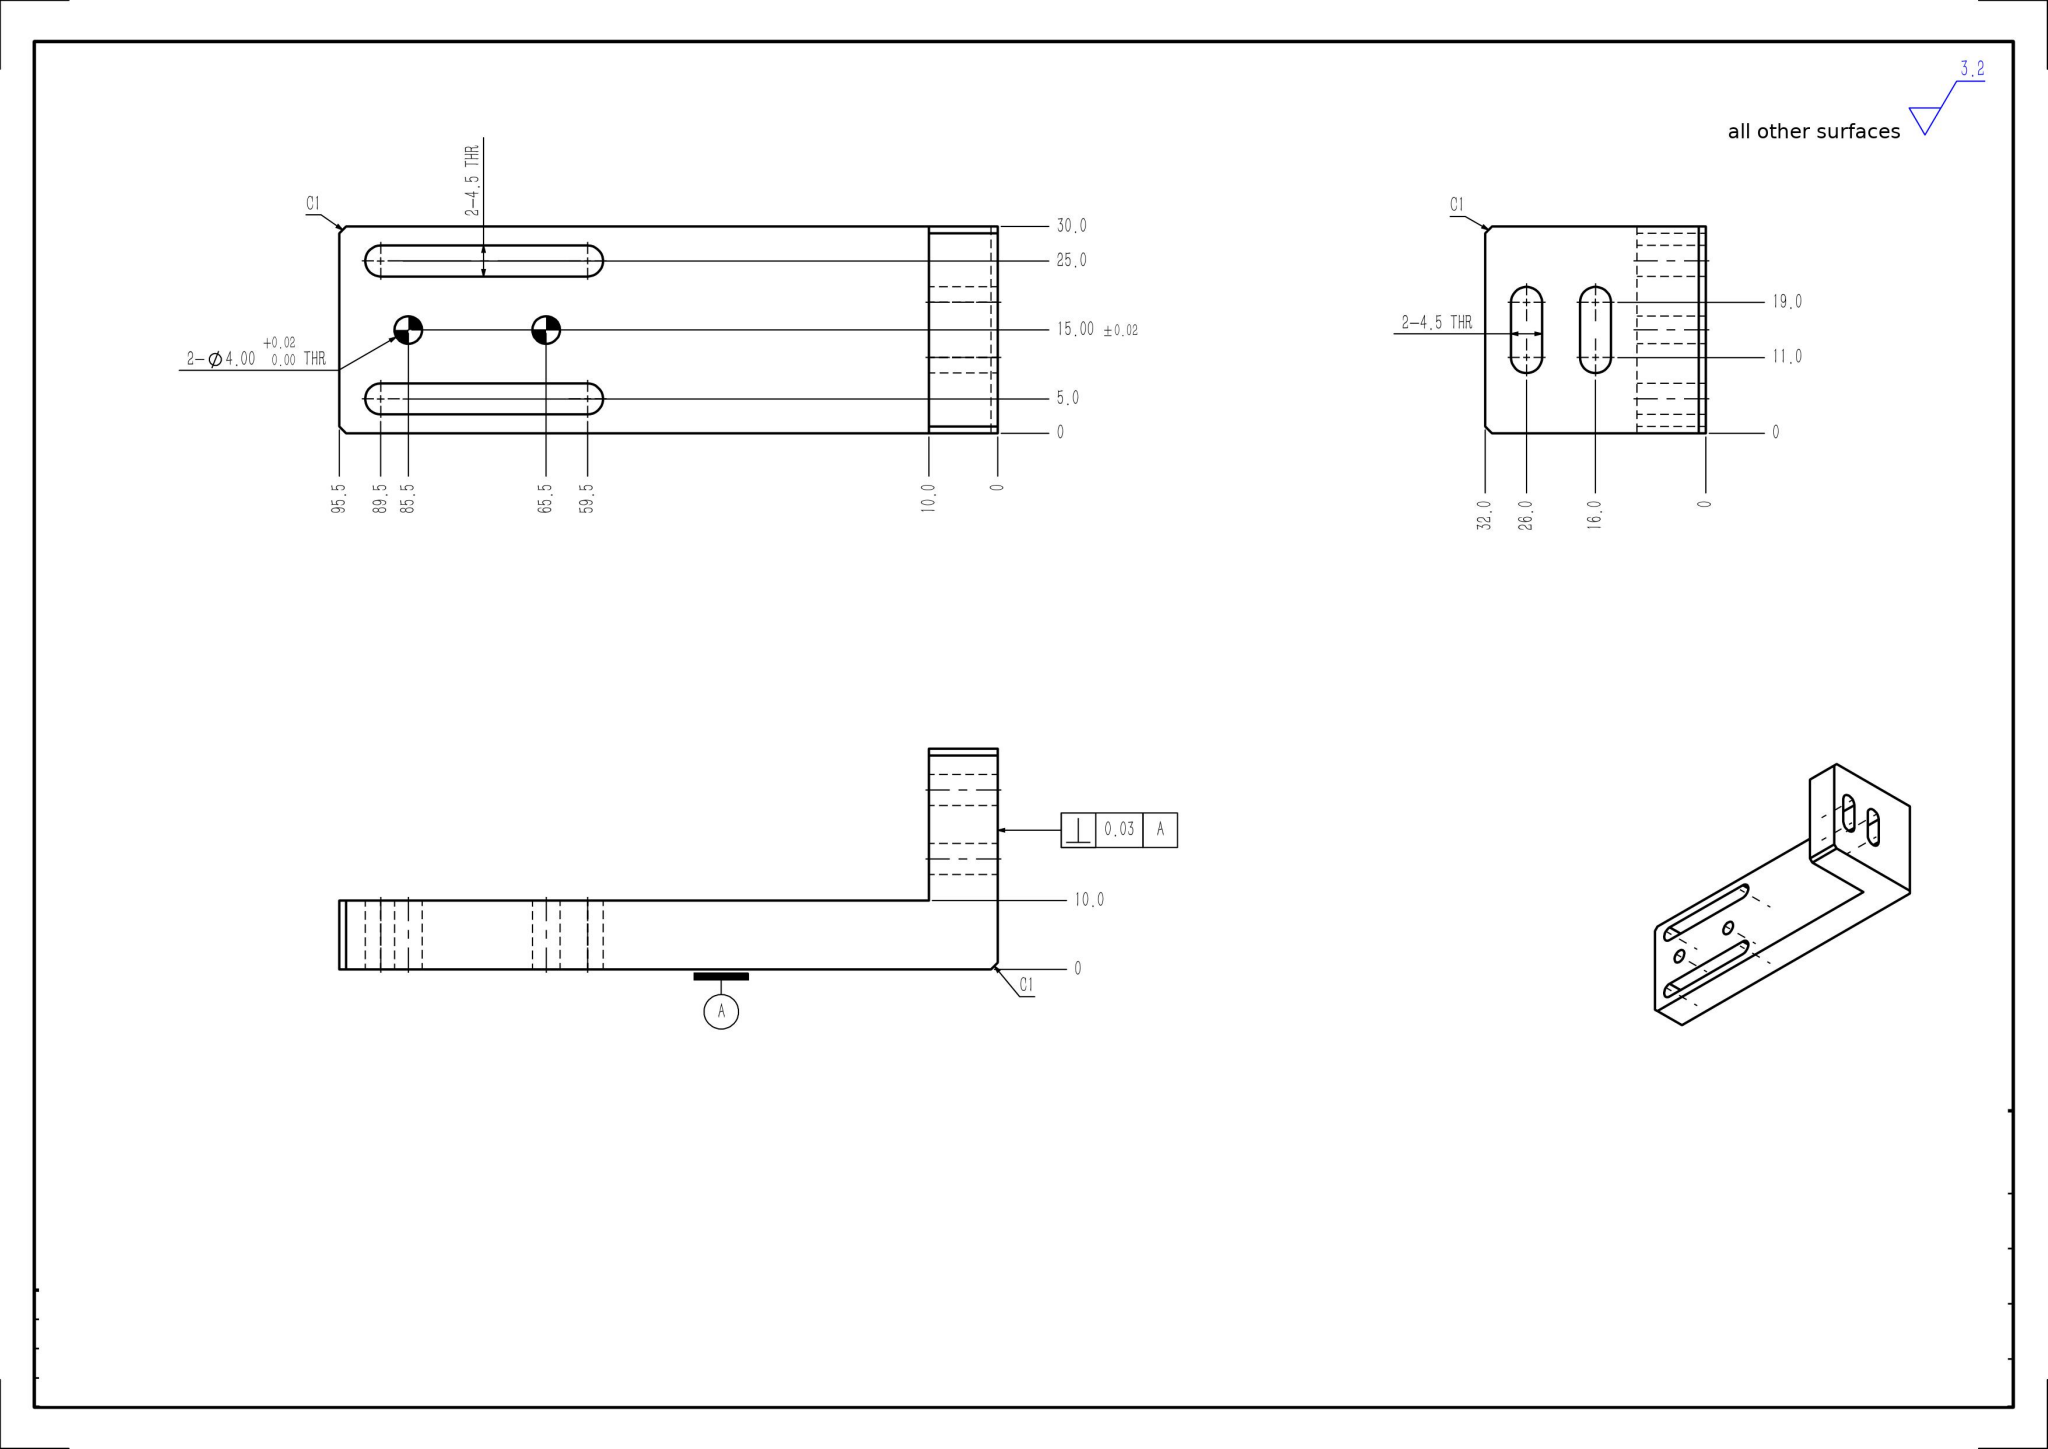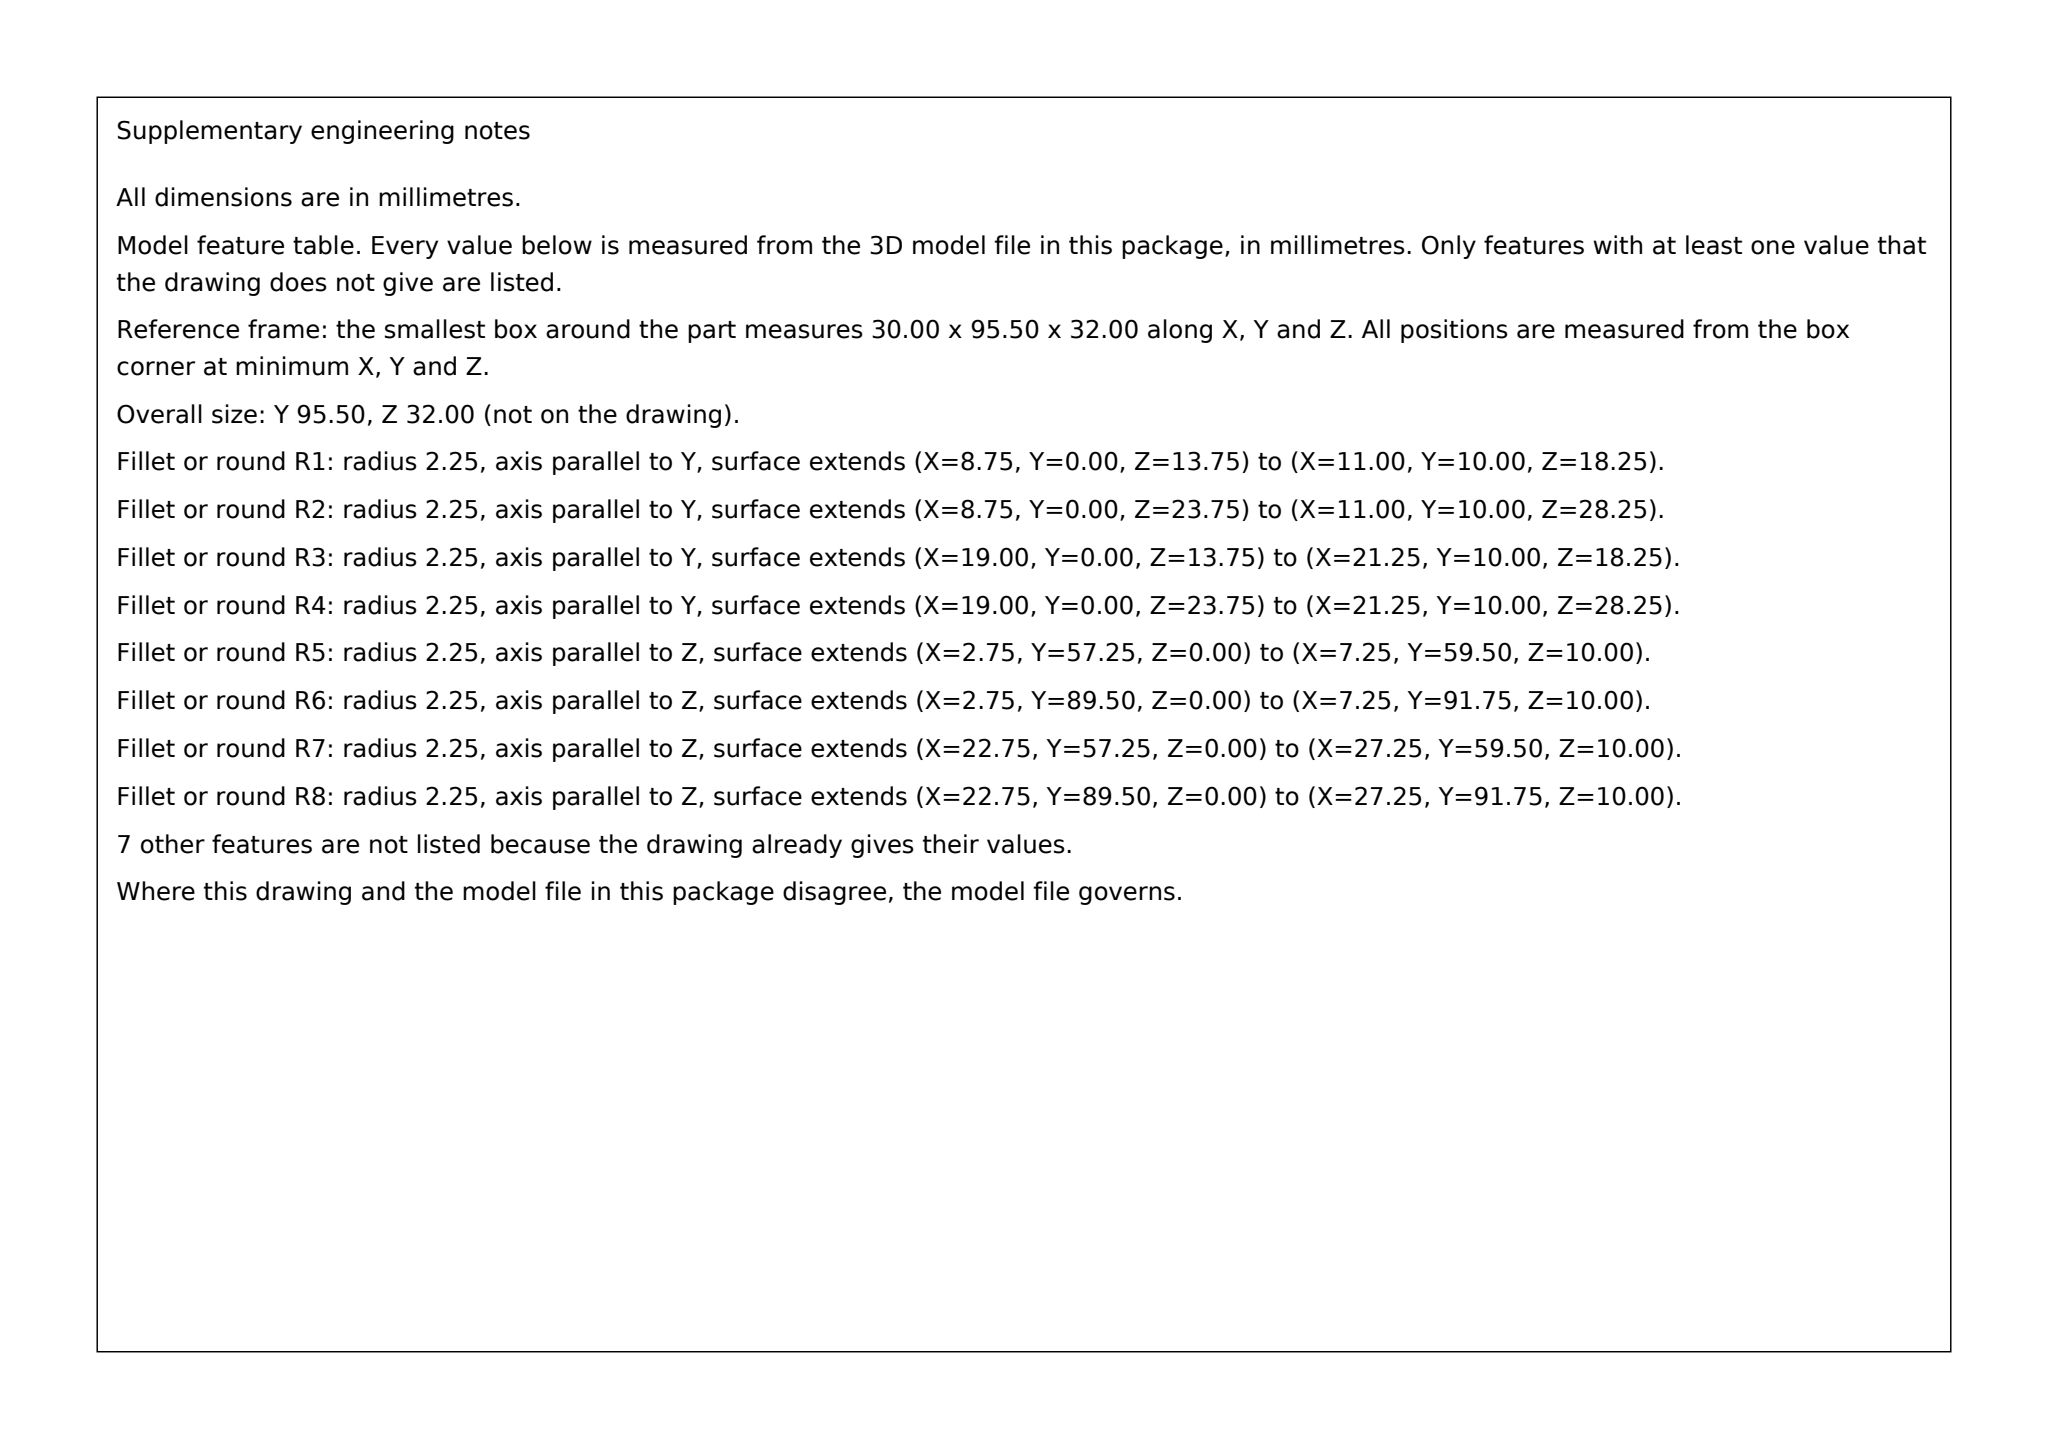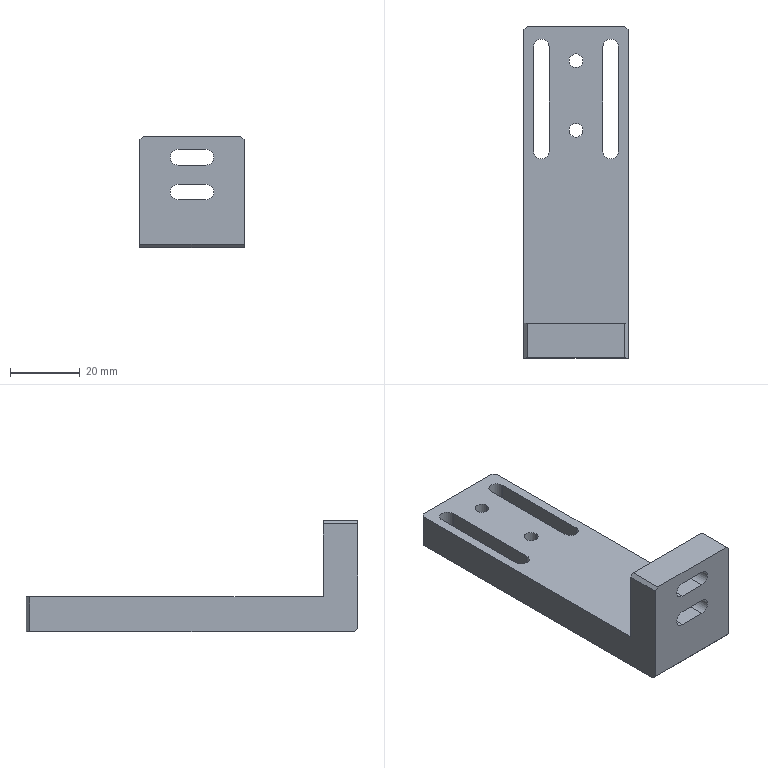Part | SolidWorks | mm | 1 solid | 33 faces | box 30 x 95.5 x 32 mm | volume 30908 mm3 | plane 21 | cylinder 12 | commonest cylinder face diameters 4.5 x8 4 x4
build123d program:
from build123d import *

# Parameters (mm, degrees)
SKETCH1_W                  = 30
SKETCH1_H                  = 95.5
BOSS_EXTRUDE1_DEPTH        = 10
SKETCH2_W                  = 30
SKETCH2_H                  = 10
BOSS_EXTRUDE2_DEPTH        = 22
M4_CLEARANCE_HOLE_1_D      = 4.5
CUT_EXTRUDE1_DEPTH         = 93.516
CUT_EXTRUDE3_DEPTH         = 55.672
SIZE_MM_DOWEL_PIN_HOLE_1_D = 4
CHAMFER1_SIZE              = 1


with BuildPart() as part:
    # Sketch1 → Boss-Extrude1 (new body)
    with BuildSketch(Plane.XY):
        Rectangle(SKETCH1_W, SKETCH1_H)
    extrude(amount=BOSS_EXTRUDE1_DEPTH)

    # Sketch2 → Boss-Extrude2 (add)
    with BuildSketch(Plane.XY.offset(10)):
        with Locations((0, -42.75)):
            Rectangle(SKETCH2_W, SKETCH2_H)
    extrude(amount=BOSS_EXTRUDE2_DEPTH)

    # M4 Clearance Hole 1 (through all)
    with Locations(Plane(origin=(0, -37.75, 0), x_dir=(1, 0, 0), z_dir=(0, 1, 0))):
        with Locations((0, -26), (0, -16)):
            Hole(M4_CLEARANCE_HOLE_1_D / 2)

    # Sketch3 → Cut-Extrude1 (cut, through all)
    with BuildSketch(Plane(origin=(0, -37.75, 0), x_dir=(1, 0, 0), z_dir=(0, 1, 0))):
        with BuildLine():
            Line((-4, -23.75), (4, -23.75))
            ThreePointArc((4, -23.75), (6.25, -26), (4, -28.25))
            Line((4, -28.25), (-4, -28.25))
            ThreePointArc((-4, -28.25), (-6.25, -26), (-4, -23.75))
        make_face()
        with BuildLine():
            Line((-4, -13.75), (4, -13.75))
            ThreePointArc((4, -13.75), (6.25, -16), (4, -18.25))
            Line((4, -18.25), (-4, -18.25))
            ThreePointArc((-4, -18.25), (-6.25, -16), (-4, -13.75))
        make_face()
    extrude(amount=-CUT_EXTRUDE1_DEPTH, mode=Mode.SUBTRACT)

    # Sketch5 → Cut-Extrude3 (cut, through all)
    with BuildSketch(Plane.XY.offset(10)):
        with BuildLine():
            Line((-7.75, 41.75), (-7.75, 11.75))
            ThreePointArc((-7.75, 11.75), (-10, 9.5), (-12.25, 11.75))
            Line((-12.25, 11.75), (-12.25, 41.75))
            ThreePointArc((-12.25, 41.75), (-10, 44), (-7.75, 41.75))
        make_face()
        with BuildLine():
            Line((12.25, 41.75), (12.25, 11.75))
            ThreePointArc((12.25, 11.75), (10, 9.5), (7.75, 11.75))
            Line((7.75, 11.75), (7.75, 41.75))
            ThreePointArc((7.75, 41.75), (10, 44), (12.25, 41.75))
        make_face()
    extrude(amount=-CUT_EXTRUDE3_DEPTH, mode=Mode.SUBTRACT)

    # Size mm Dowel Pin Hole 1 (through all)
    with Locations(Plane.XY.offset(10)):
        with Locations((0, 37.75), (0, 17.75)):
            Hole(SIZE_MM_DOWEL_PIN_HOLE_1_D / 2)

    # Chamfer1
    chamfer1_edges = [part.edges().sort_by_distance(p)[0] for p in [
        (-15, -42.75, 32),
        (15, -42.75, 32),
        (0, -47.75, 0),
        (-15, 47.75, 5),
        (15, 47.75, 5),
    ]]
    chamfer(chamfer1_edges, length=CHAMFER1_SIZE)


solid = part.part